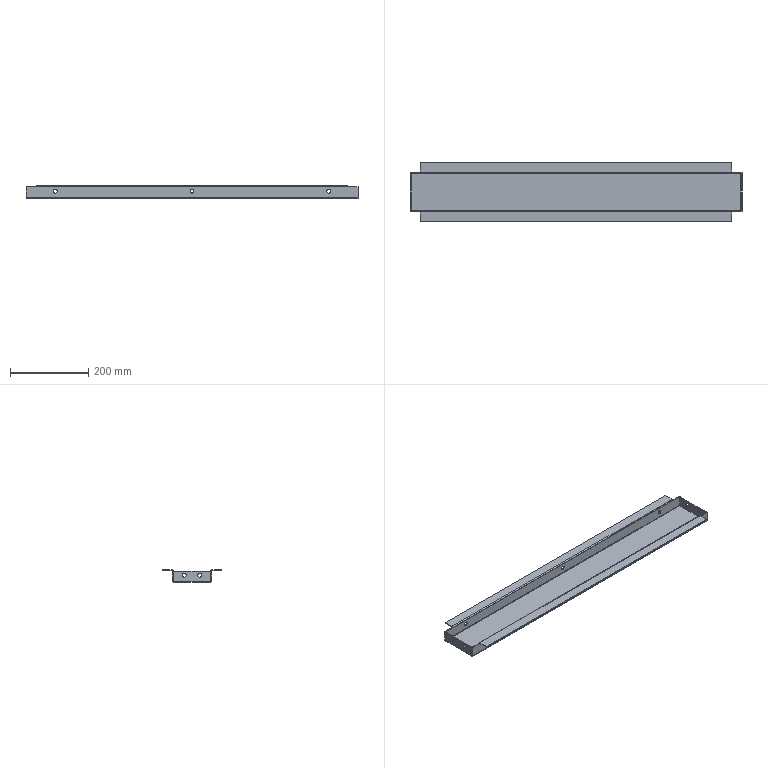Component | SolidWorks | 30RearMiddleBeamII-1 | 1 solid | 82 faces | volume 353400 mm3 | plane 50 | cylinder 32 | commonest cylinder face diameters 10 x20 6 x6 2 x6